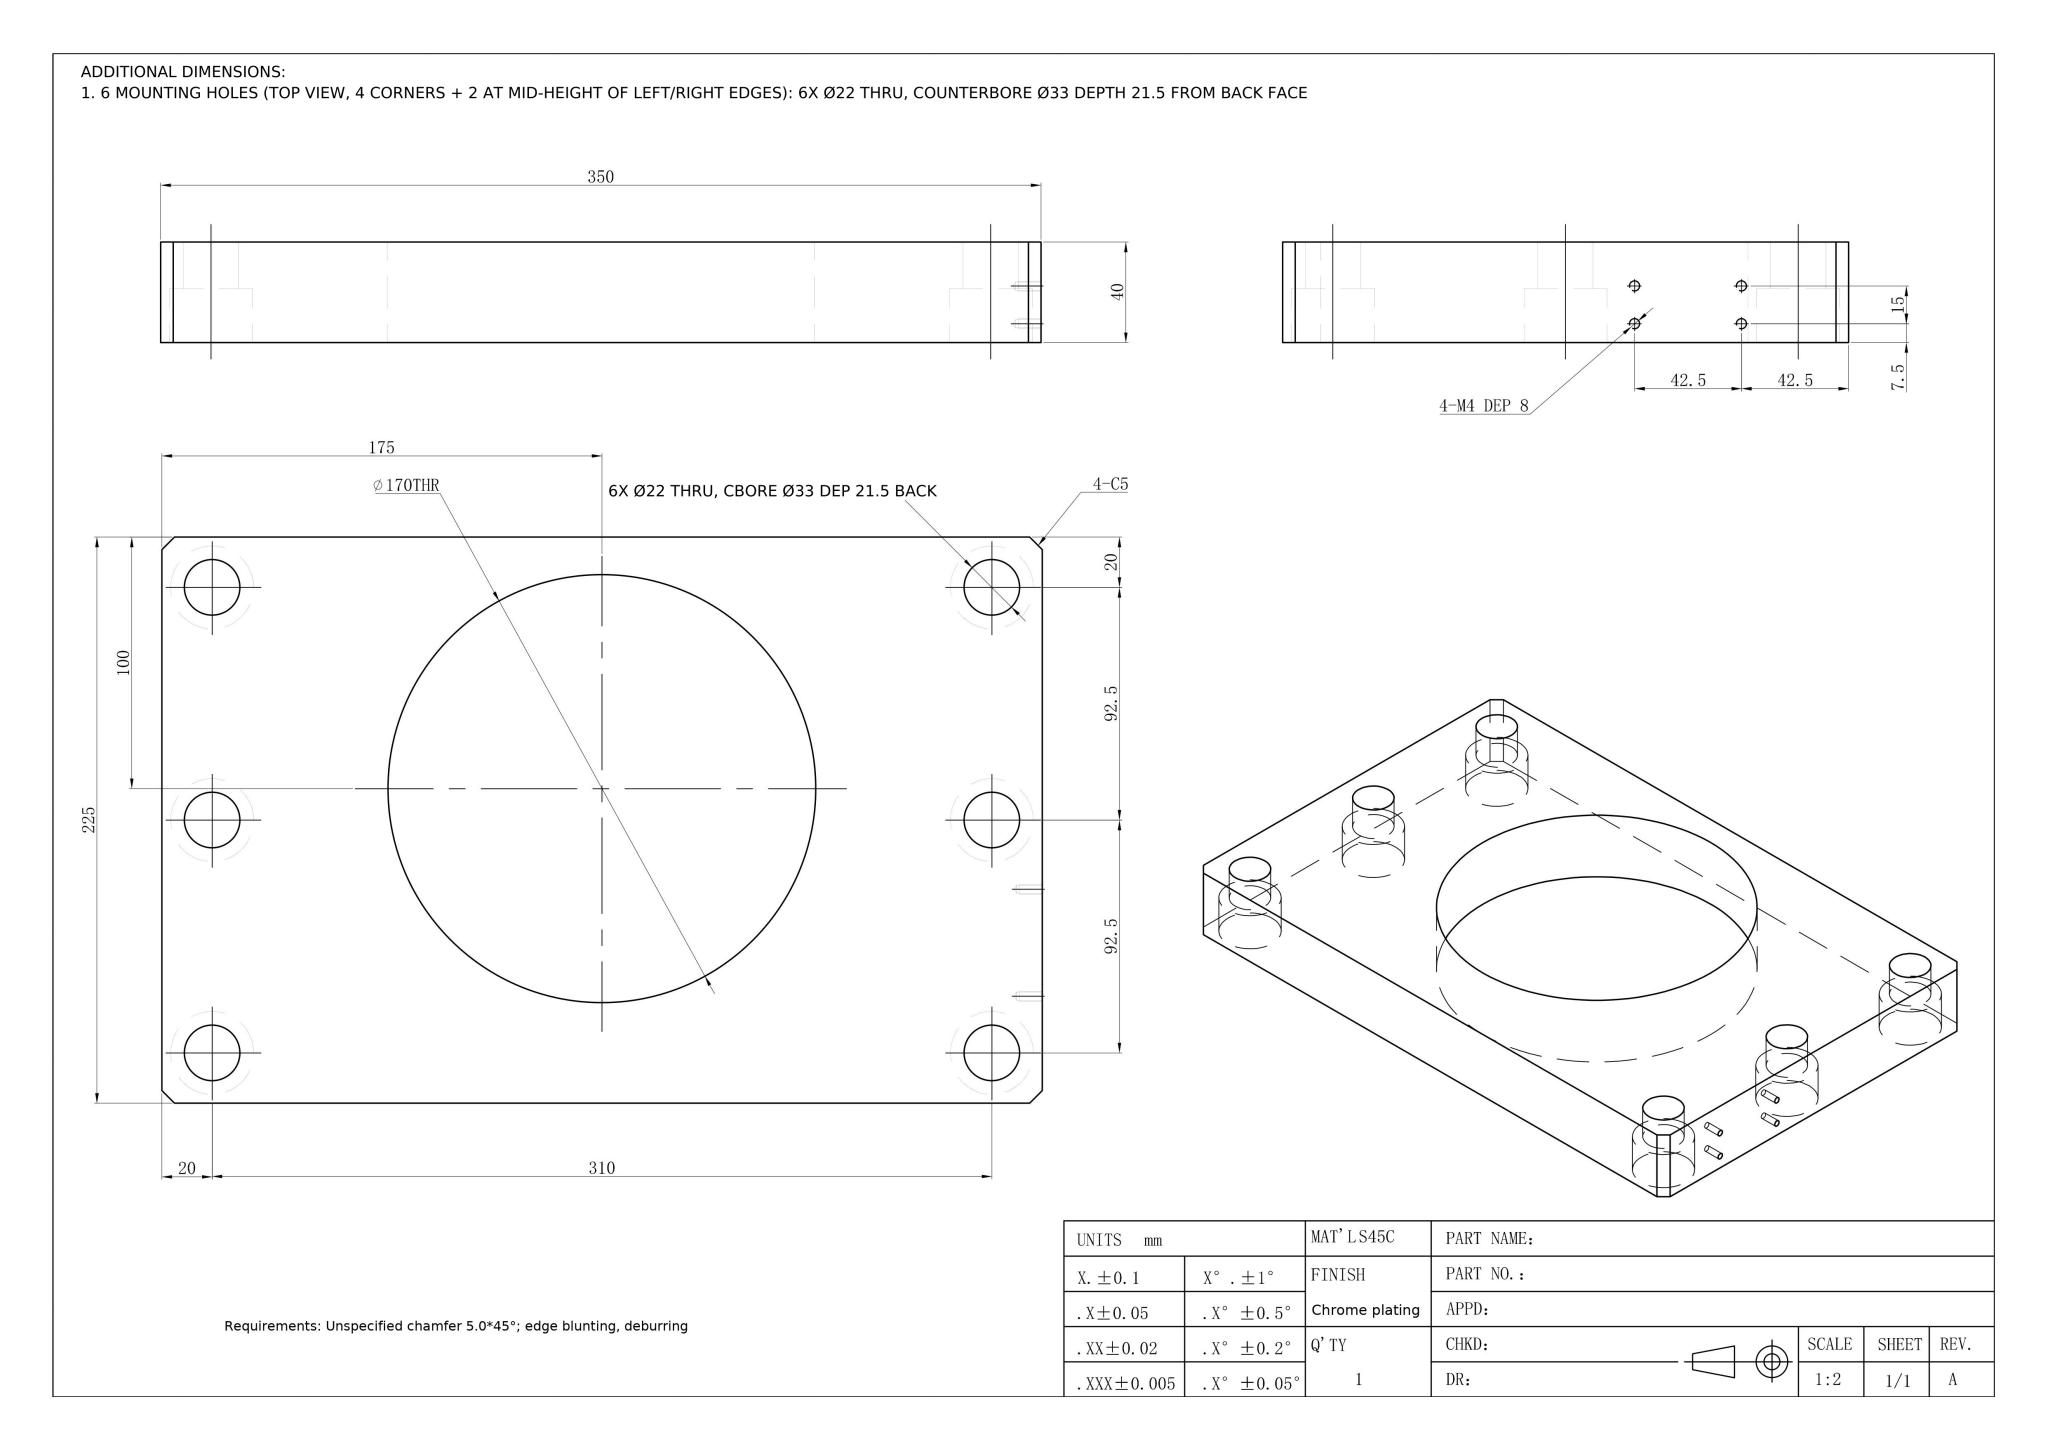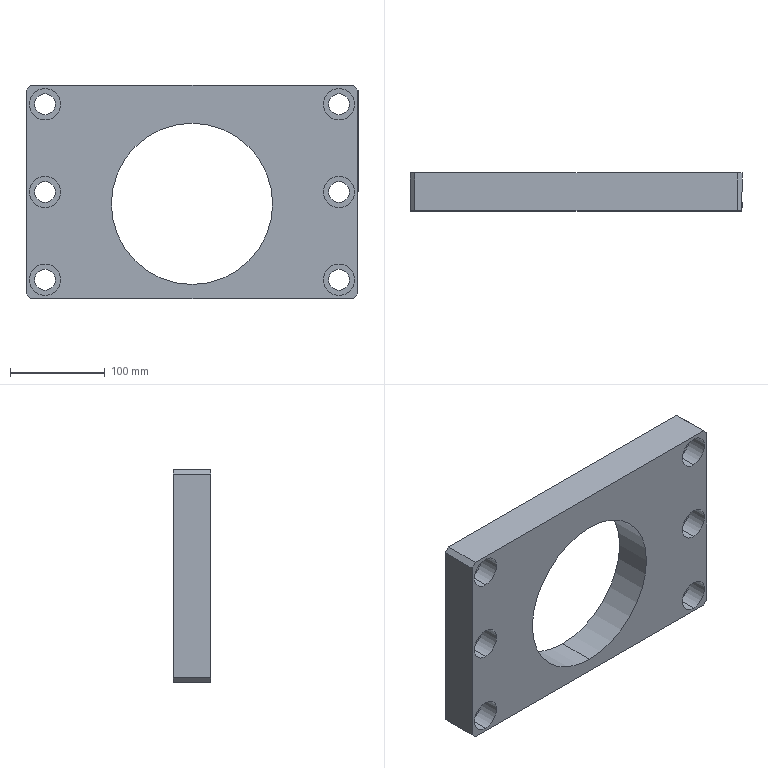Part | NX | mm | 1 solid | 58 faces | box 350 x 40 x 225 mm | volume 2087195 mm3 | cylinder 34 | plane 16 | cone 8 | commonest cylinder face diameters 22 x12 33 x12 3.3 x8 170 x2